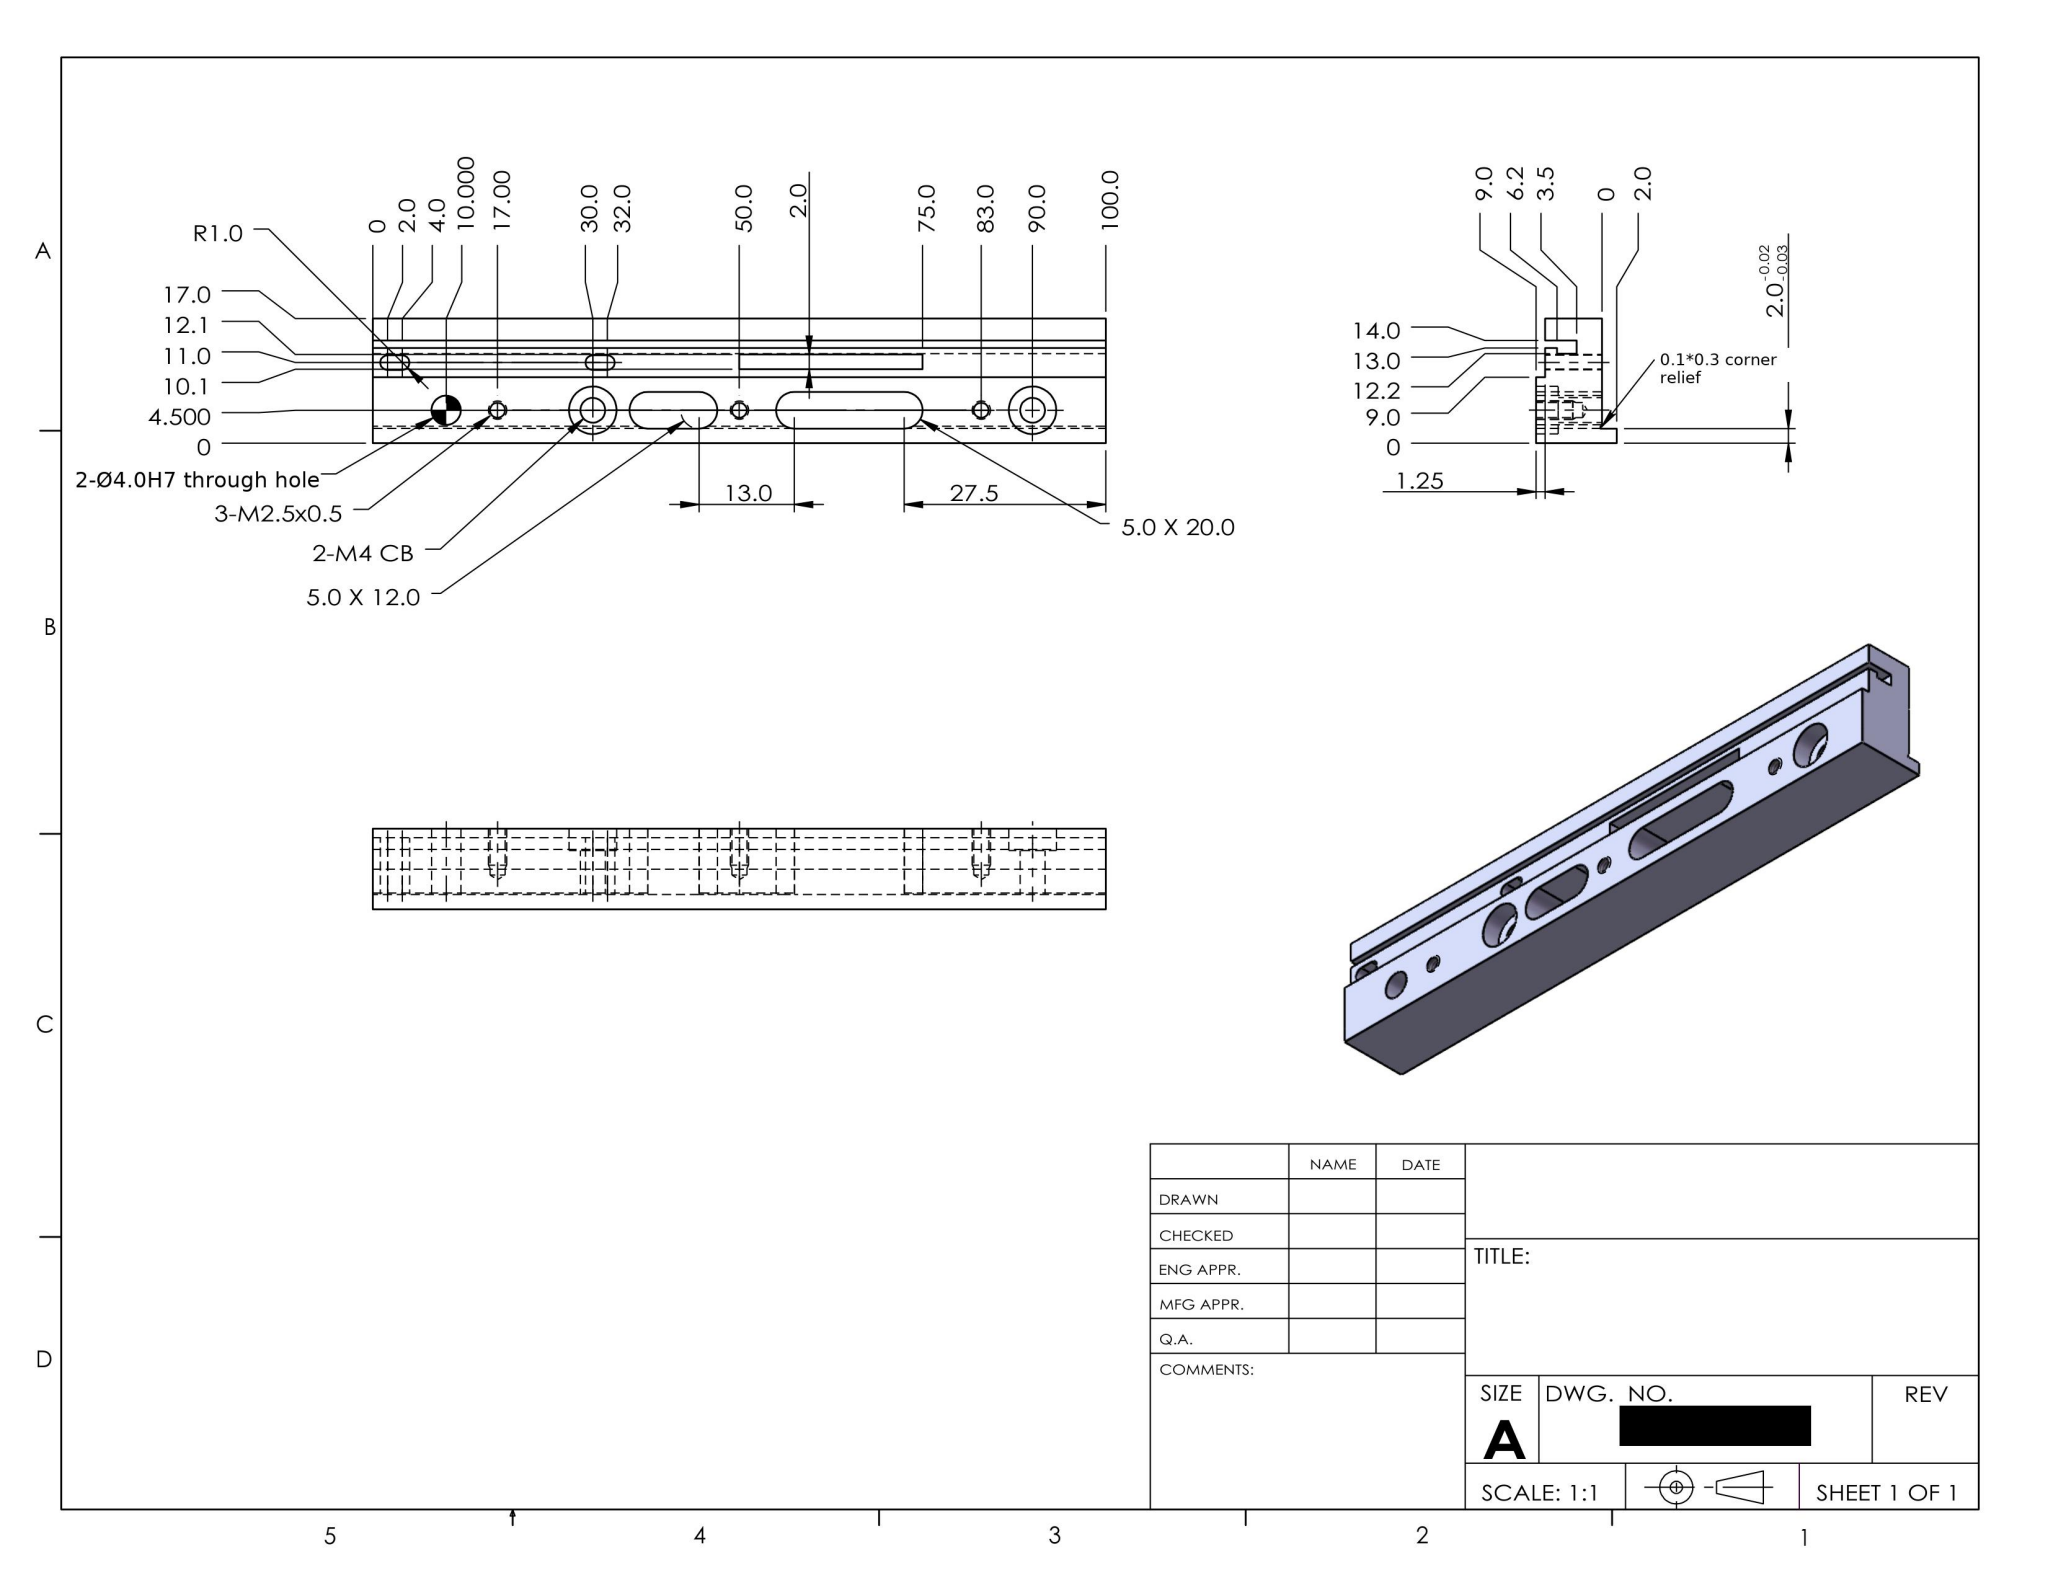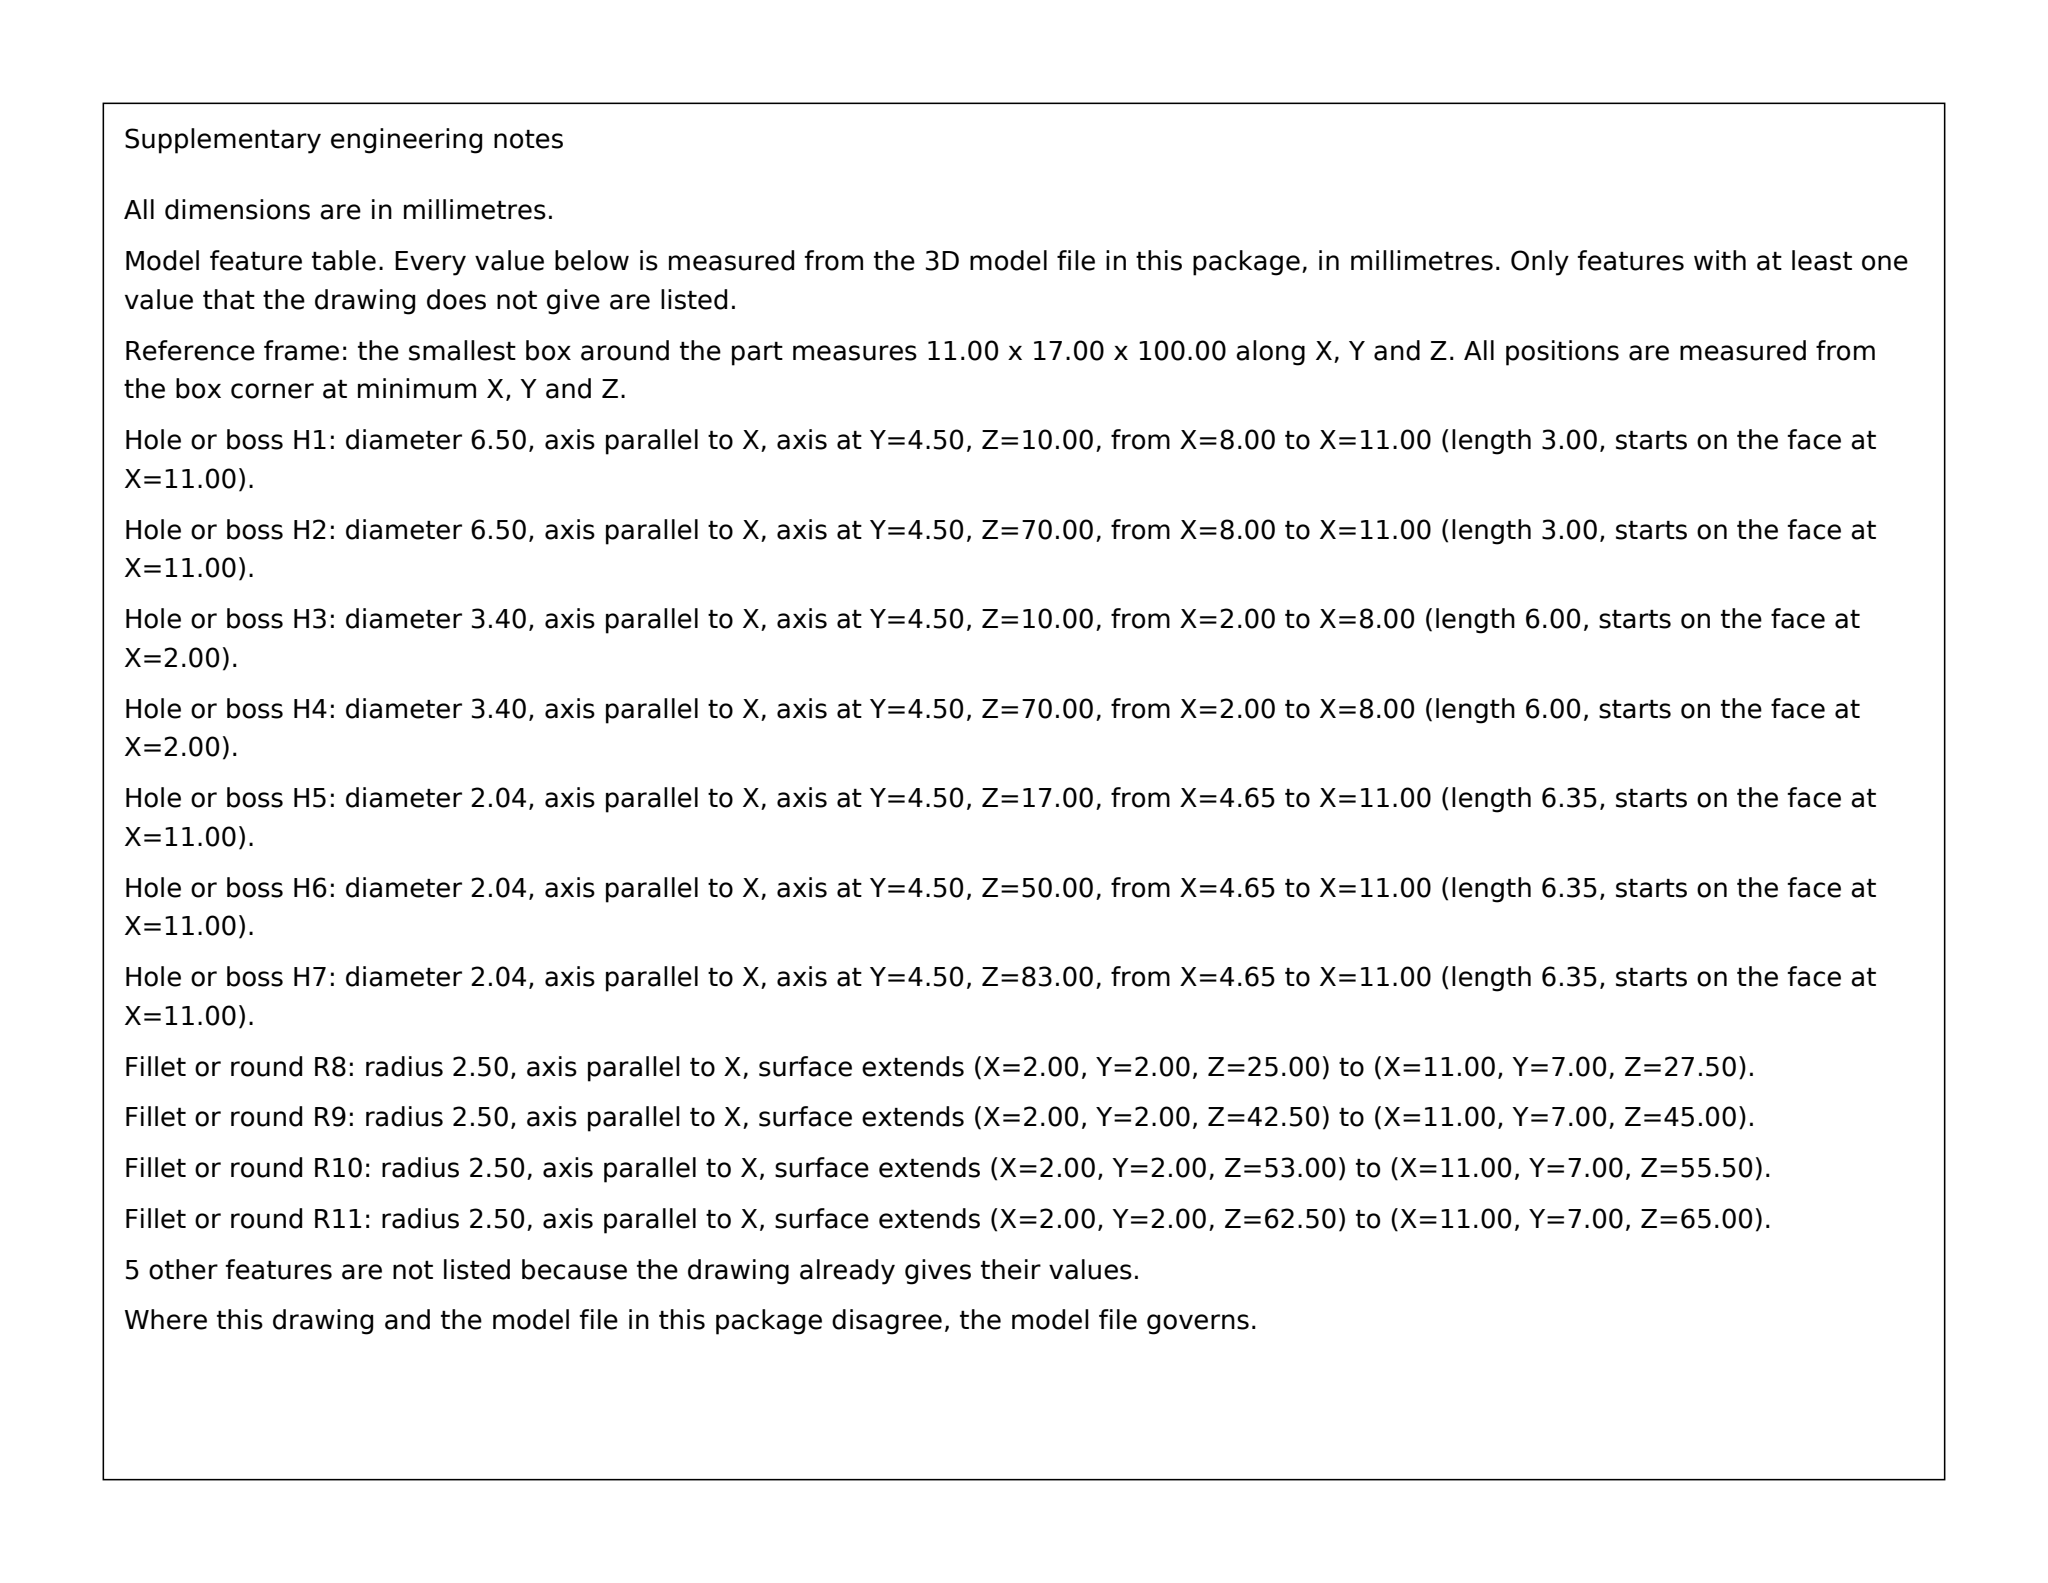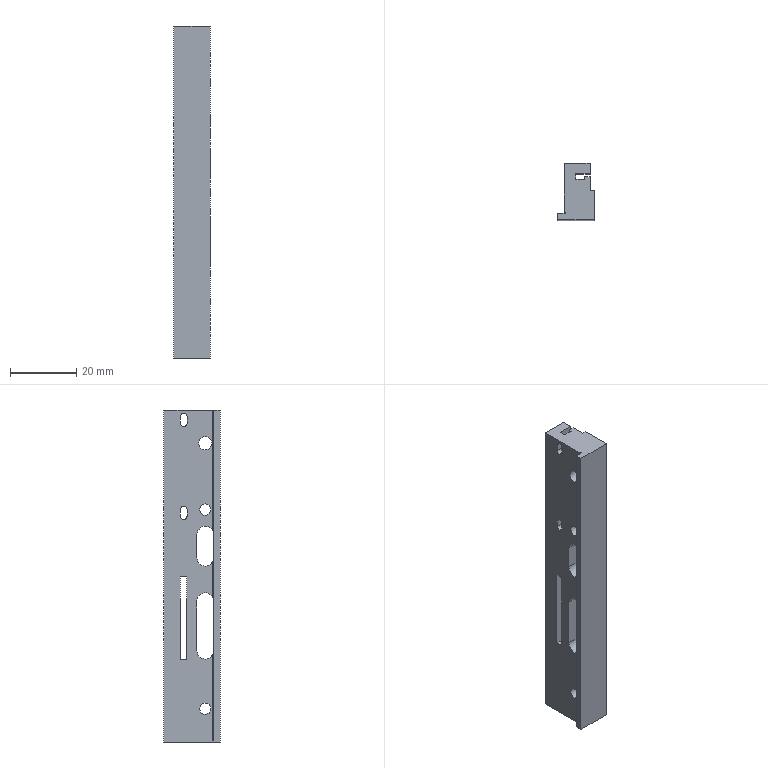Part | SolidWorks | mm | 1 solid | 68 faces | box 11 x 17 x 100 mm | volume 11722 mm3 | plane 34 | cylinder 28 | cone 6 | commonest cylinder face diameters 5 x6 2.05 x6 2 x6 6.5 x4 3.4 x4 4 x2
build123d program:
from build123d import *

# Parameters (mm, degrees)
SKETCH1_W                                            = 240
SKETCH1_H                                            = 30
EXTRUDE1_DEPTH                                       = 9
SKETCH2_W                                            = 240
SKETCH2_H                                            = 8
EXTRUDE2_DEPTH                                       = 1.25
SKETCH3_W                                            = 4.3
SKETCH3_H                                            = 1
EXTRUDE3_DEPTH                                       = 243.035
SKETCH5_W                                            = 9
SKETCH5_H                                            = 9
CUT_EXTRUDE1_DEPTH                                   = 243.035
CHAMFER1_SIZE                                        = 0.5
CHAMFER1_SIZE2                                       = 3
CHAMFER2_SIZE                                        = 3
CHAMFER2_SIZE2                                       = 0.5
CHAMFER3_SIZE                                        = 0.3
CHAMFER3_SIZE2                                       = 3
CYLINDRICAL_COUNTERSUNK_HOLE_FOR_M3_SOCK_D           = 3.4
CYLINDRICAL_COUNTERSUNK_HOLE_FOR_M3_SOCK_CBORE_D     = 6.5
CYLINDRICAL_COUNTERSUNK_HOLE_FOR_M3_SOCK_CBORE_DEPTH = 3
LPATTERN1_COUNT                                      = 4
LPATTERN1_PITCH                                      = 60
SKETCH8_W                                            = 2
SKETCH8_H                                            = 2
EXTRUDE5_DEPTH                                       = 240
SKETCH9_W                                            = 0.2
SKETCH9_H                                            = 0.3
EXTRUDE6_DEPTH                                       = 242.085
SKETCH10_W                                           = 9
SKETCH10_H                                           = 4
EXTRUDE7_DEPTH                                       = 242.085
SKETCH11_R                                           = 2
CUT_EXTRUDE2_DEPTH                                   = 241.853
SKETCH12_W                                           = 2.7
SKETCH12_H                                           = 0.8
EXTRUDE8_DEPTH                                       = 241.77
SKETCH13_W                                           = 25
SKETCH13_H                                           = 2
CUT_EXTRUDE3_DEPTH                                   = 241.799
SKETCH15_R                                           = 0.75
CUT_EXTRUDE4_DEPTH                                   = 241.799
EXTRUDE9_DEPTH                                       = 241.799
SKETCH17_W                                           = 15
SKETCH17_H                                           = 9
CUT_EXTRUDE5_DEPTH                                   = 1.2
M2_5X0_45_TAPPED_HOLE1_D                             = 2.05
M2_5X0_45_TAPPED_HOLE1_DEPTH                         = 6.35
M2_5X0_45_TAPPED_HOLE1_TIP                           = 0.6159
SKETCH20_W                                           = 5
SKETCH20_H                                           = 3
CUT_EXTRUDE6_DEPTH                                   = 241.799
FILLET1_R                                            = 0.3
SKETCH21_OUTSIDE_W                                   = 290.17
SKETCH21_OUTSIDE_H                                   = 67.17
SKETCH21_OUTSIDE_W_2                                 = 100
SKETCH21_OUTSIDE_H_2                                 = 17
EXTRUDE10_DEPTH                                      = 241.853
CUT_EXTRUDE7_DEPTH                                   = 103.029


with BuildPart() as part:
    # Sketch1 → Extrude1 (new body)
    with BuildSketch(Plane(origin=(0, 0, 0), x_dir=(0, 0, -1), z_dir=(1, 0, 0))):
        with Locations((120, 15)):
            Rectangle(SKETCH1_W, SKETCH1_H)
    extrude(amount=EXTRUDE1_DEPTH)

    # Sketch2 → Extrude2 (cut)
    with BuildSketch(Plane(origin=(9, 0, 0), x_dir=(0, 0, -1), z_dir=(1, 0, 0))):
        with Locations((120, 13)):
            Rectangle(SKETCH2_W, SKETCH2_H)
    extrude(amount=-EXTRUDE2_DEPTH, mode=Mode.SUBTRACT)

    # Sketch3 → Extrude3 (cut, through all)
    with BuildSketch(Plane(origin=(0, 0, -240), x_dir=(-1, 0, 0), z_dir=(0, 0, -1))):
        with Locations((-5.6, 13.5)):
            Rectangle(SKETCH3_W, SKETCH3_H)
    extrude(amount=-EXTRUDE3_DEPTH, mode=Mode.SUBTRACT)

    # Sketch5 → Cut-Extrude1 (cut, through all)
    with BuildSketch(Plane(origin=(0, 0, -240), x_dir=(-1, 0, 0), z_dir=(0, 0, -1))):
        with Locations((-4.5, 25.5)):
            Rectangle(SKETCH5_W, SKETCH5_H)
    extrude(amount=-CUT_EXTRUDE1_DEPTH, mode=Mode.SUBTRACT)

    # Chamfer1
    chamfer1_edges = [part.edges().sort_by_distance(p)[0] for p in [
        (7.75, 11, -240),
        (7.75, 15.5, -240),
    ]]
    chamfer1_side = [part.faces().sort_by_distance(p)[0] for p in [
        (4.251, 10.283, -240),
    ]]
    chamfer(chamfer1_edges, length=CHAMFER1_SIZE, length2=CHAMFER1_SIZE2, reference=chamfer1_side[0])

    # Chamfer2
    chamfer2_edges = [part.edges().sort_by_distance(p)[0] for p in [
        (8.125, 9, -240),
    ]]
    chamfer2_side = [part.faces().sort_by_distance(p)[0] for p in [
        (8.373, 9, -120.297),
    ]]
    chamfer(chamfer2_edges, length=CHAMFER2_SIZE, length2=CHAMFER2_SIZE2, reference=chamfer2_side[0])

    # Chamfer3
    chamfer3_edges = [part.edges().sort_by_distance(p)[0] for p in [
        (5.35, 14, -240),
        (5.35, 13, -240),
    ]]
    chamfer3_side = [part.faces().sort_by_distance(p)[0] for p in [
        (4.164, 10.237, -240),
    ]]
    chamfer(chamfer3_edges, length=CHAMFER3_SIZE, length2=CHAMFER3_SIZE2, reference=chamfer3_side[0])

    # Cylindrical Countersunk Hole for M3 Sock (through all)
    with Locations(Plane(origin=(9, 0, 0), x_dir=(0, 0, -1), z_dir=(1, 0, 0))):
        with Locations((30, 4.5)):
            cylindrical_countersunk_hole_for_m3_sock = CounterBoreHole(CYLINDRICAL_COUNTERSUNK_HOLE_FOR_M3_SOCK_D / 2, CYLINDRICAL_COUNTERSUNK_HOLE_FOR_M3_SOCK_CBORE_D / 2, CYLINDRICAL_COUNTERSUNK_HOLE_FOR_M3_SOCK_CBORE_DEPTH)

    # LPattern1: Cylindrical Countersunk Hole for M3 Sock ×4
    with Locations(*[(0, 0, -i * LPATTERN1_PITCH) for i in range(1, LPATTERN1_COUNT)]):
        add(cylindrical_countersunk_hole_for_m3_sock, mode=Mode.SUBTRACT)

    # Sketch8 → Extrude5 (add)
    with BuildSketch(Plane(origin=(0, 0, -240), x_dir=(-1, 0, 0), z_dir=(0, 0, -1))):
        with Locations((1, 1)):
            Rectangle(SKETCH8_W, SKETCH8_H)
    extrude(amount=-EXTRUDE5_DEPTH)

    # Sketch9 → Extrude6 (cut, through all)
    with BuildSketch(Plane(origin=(0, 0, -240), x_dir=(-1, 0, 0), z_dir=(0, 0, -1))):
        with Locations((-0.1, 2.15)):
            Rectangle(SKETCH9_W, SKETCH9_H)
    extrude(amount=-EXTRUDE6_DEPTH, mode=Mode.SUBTRACT)

    # Sketch10 → Extrude7 (cut, through all)
    with BuildSketch(Plane(origin=(0, 0, -240), x_dir=(-1, 0, 0), z_dir=(0, 0, -1))):
        with Locations((-4.5, 19)):
            Rectangle(SKETCH10_W, SKETCH10_H)
    extrude(amount=-EXTRUDE7_DEPTH, mode=Mode.SUBTRACT)

    # Sketch11 → Cut-Extrude2 (cut, through all)
    with BuildSketch(Plane(origin=(9, 0, 0), x_dir=(0, 0, -1), z_dir=(1, 0, 0))):
        with Locations((10, 4.5)):
            Circle(SKETCH11_R)
    extrude(amount=-CUT_EXTRUDE2_DEPTH, mode=Mode.SUBTRACT)

    # Sketch12 → Extrude8 (cut, through all)
    with BuildSketch(Plane.XY):
        with Locations((4.8, 12.6)):
            Rectangle(SKETCH12_W, SKETCH12_H)
    extrude(amount=-EXTRUDE8_DEPTH, mode=Mode.SUBTRACT)

    # Sketch13 → Cut-Extrude3 (cut, through all)
    with BuildSketch(Plane(origin=(7.75, 0, 0), x_dir=(0, 0, -1), z_dir=(1, 0, 0))):
        with Locations((62.5, 11.1)):
            Rectangle(SKETCH13_W, SKETCH13_H)
    extrude(amount=-CUT_EXTRUDE3_DEPTH, mode=Mode.SUBTRACT)

    # Sketch15 → Cut-Extrude4 (cut, through all)
    with BuildSketch(Plane(origin=(7.75, 0, 0), x_dir=(0, 0, -1), z_dir=(1, 0, 0))):
        with Locations((3, 11)):
            Circle(SKETCH15_R)
        with Locations((31, 11)):
            Circle(SKETCH15_R)
    extrude(amount=-CUT_EXTRUDE4_DEPTH, mode=Mode.SUBTRACT)

    # Sketch16 → Extrude9 (cut, through all)
    with BuildSketch(Plane(origin=(7.75, 0, 0), x_dir=(0, 0, -1), z_dir=(1, 0, 0))):
        with BuildLine():
            Line((2, 12), (4, 12))
            ThreePointArc((4, 12), (5, 11), (4, 10))
            Line((4, 10), (2, 10))
            ThreePointArc((2, 10), (1, 11), (2, 12))
        make_face()
        with BuildLine():
            Line((32, 10), (30, 10))
            ThreePointArc((30, 10), (29, 11), (30, 12))
            Line((30, 12), (32, 12))
            ThreePointArc((32, 12), (33, 11), (32, 10))
        make_face()
    extrude(amount=-EXTRUDE9_DEPTH, mode=Mode.SUBTRACT)

    # Sketch17 → Cut-Extrude5 (cut)
    with BuildSketch(Plane(origin=(9, 0, 0), x_dir=(0, 0, -1), z_dir=(1, 0, 0))):
        with Locations((172.5, 4.5)):
            Rectangle(SKETCH17_W, SKETCH17_H)
    extrude(amount=-CUT_EXTRUDE5_DEPTH, mode=Mode.SUBTRACT)

    # M2.5x0.45 Tapped Hole1
    with Locations(Plane(origin=(9, 0, 0), x_dir=(0, 0, -1), z_dir=(1, 0, 0))):
        with Locations((230, 4.5), (200, 4.5), (140, 4.5), (110, 4.5), (83, 4.5), (50, 4.5), (17, 4.5)):
            Hole(M2_5X0_45_TAPPED_HOLE1_D / 2, depth=M2_5X0_45_TAPPED_HOLE1_DEPTH)
            with Locations((0, 0, -(M2_5X0_45_TAPPED_HOLE1_DEPTH + M2_5X0_45_TAPPED_HOLE1_TIP / 2))):  # 118° drill point
                Cone(0, M2_5X0_45_TAPPED_HOLE1_D / 2, M2_5X0_45_TAPPED_HOLE1_TIP, mode=Mode.SUBTRACT)

    # Sketch20 → Cut-Extrude6 (cut, through all)
    with BuildSketch(Plane(origin=(7.75, 0, 0), x_dir=(0, 0, -1), z_dir=(1, 0, 0))):
        with Locations((123, 11)):
            Rectangle(SKETCH20_W, SKETCH20_H)
    extrude(amount=-CUT_EXTRUDE6_DEPTH, mode=Mode.SUBTRACT)

    # Fillet1
    fillet1_edges = [part.edges().sort_by_distance(p)[0] for p in [
        (1.725, 12.5, -120.5),
        (1.725, 12.5, -125.5),
        (3.875, 9.5, -125.5),
        (3.875, 9.5, -120.5),
    ]]
    fillet(fillet1_edges, radius=FILLET1_R)

    # Sketch21 outside → Extrude10 (cut, through all)
    with BuildSketch(Plane(origin=(9, 0, 0), x_dir=(0, 0, -1), z_dir=(1, 0, 0))):
        with Locations((120, 8.5)):
            Rectangle(SKETCH21_OUTSIDE_W, SKETCH21_OUTSIDE_H)
        with Locations((50, 8.5)):
            Rectangle(SKETCH21_OUTSIDE_W_2, SKETCH21_OUTSIDE_H_2, mode=Mode.SUBTRACT)
    extrude(amount=-EXTRUDE10_DEPTH, mode=Mode.SUBTRACT)

    # Sketch22 → Cut-Extrude7 (cut, through all)
    with BuildSketch(Plane(origin=(9, 0, 0), x_dir=(0, 0, -1), z_dir=(1, 0, 0))):
        with BuildLine():
            Line((57.5, 7), (72.5, 7))
            ThreePointArc((72.5, 7), (75, 4.5), (72.5, 2))
            Line((72.5, 2), (57.5, 2))
            ThreePointArc((57.5, 2), (55, 4.5), (57.5, 7))
        make_face()
        with BuildLine():
            Line((37.5, 7), (44.5, 7))
            ThreePointArc((44.5, 7), (47, 4.5), (44.5, 2))
            Line((44.5, 2), (37.5, 2))
            ThreePointArc((37.5, 2), (35, 4.5), (37.5, 7))
        make_face()
    extrude(amount=-CUT_EXTRUDE7_DEPTH, mode=Mode.SUBTRACT)


solid = part.part